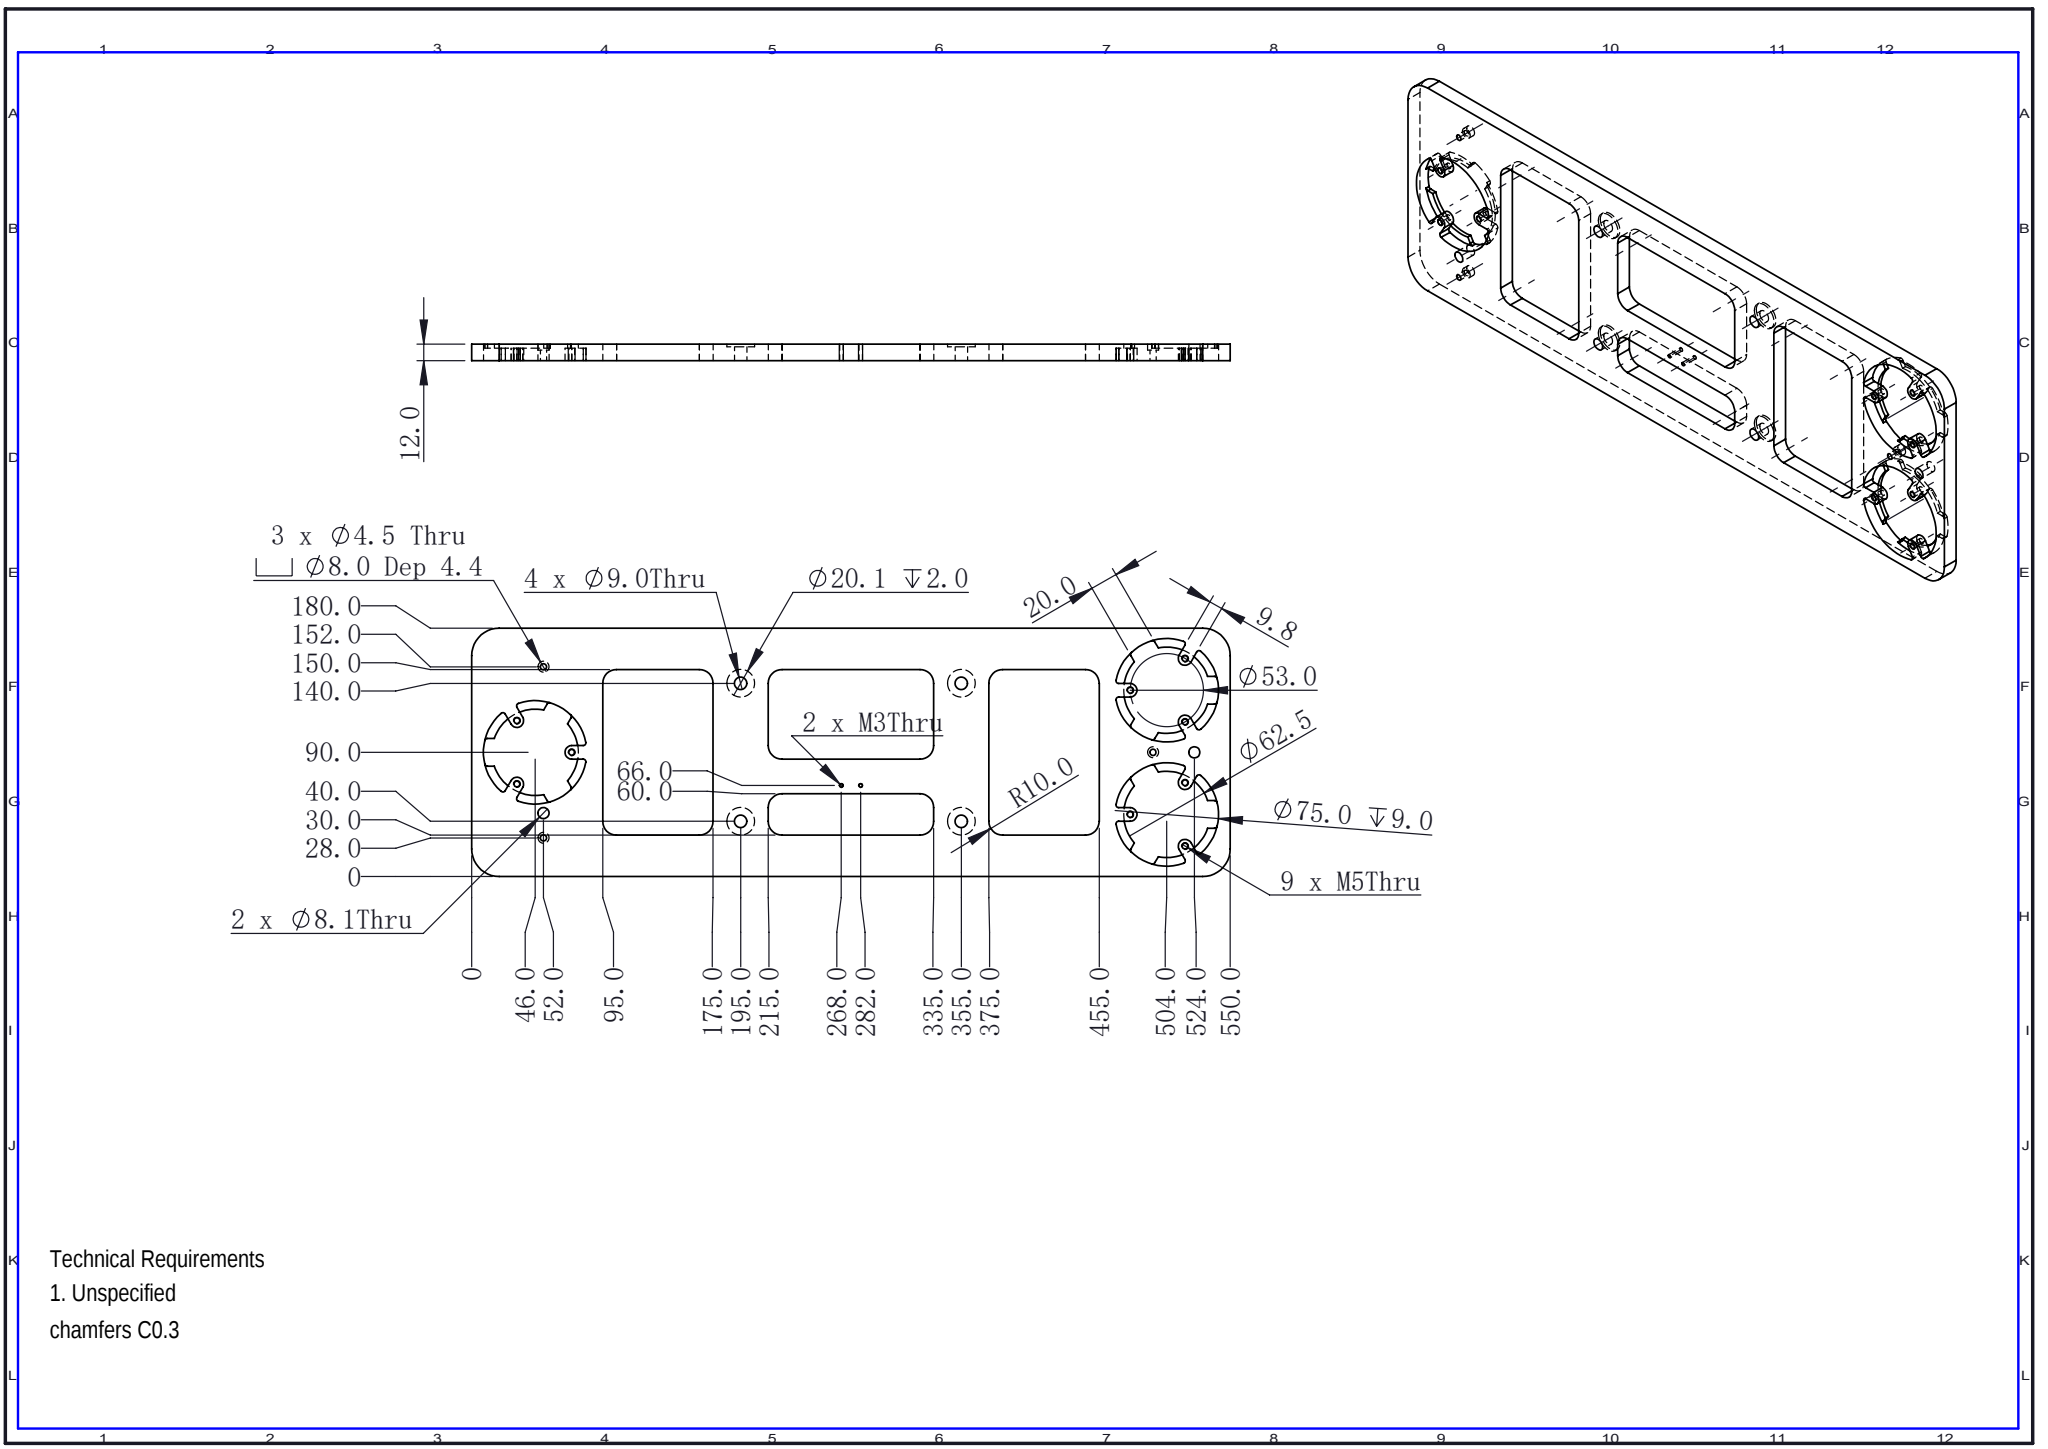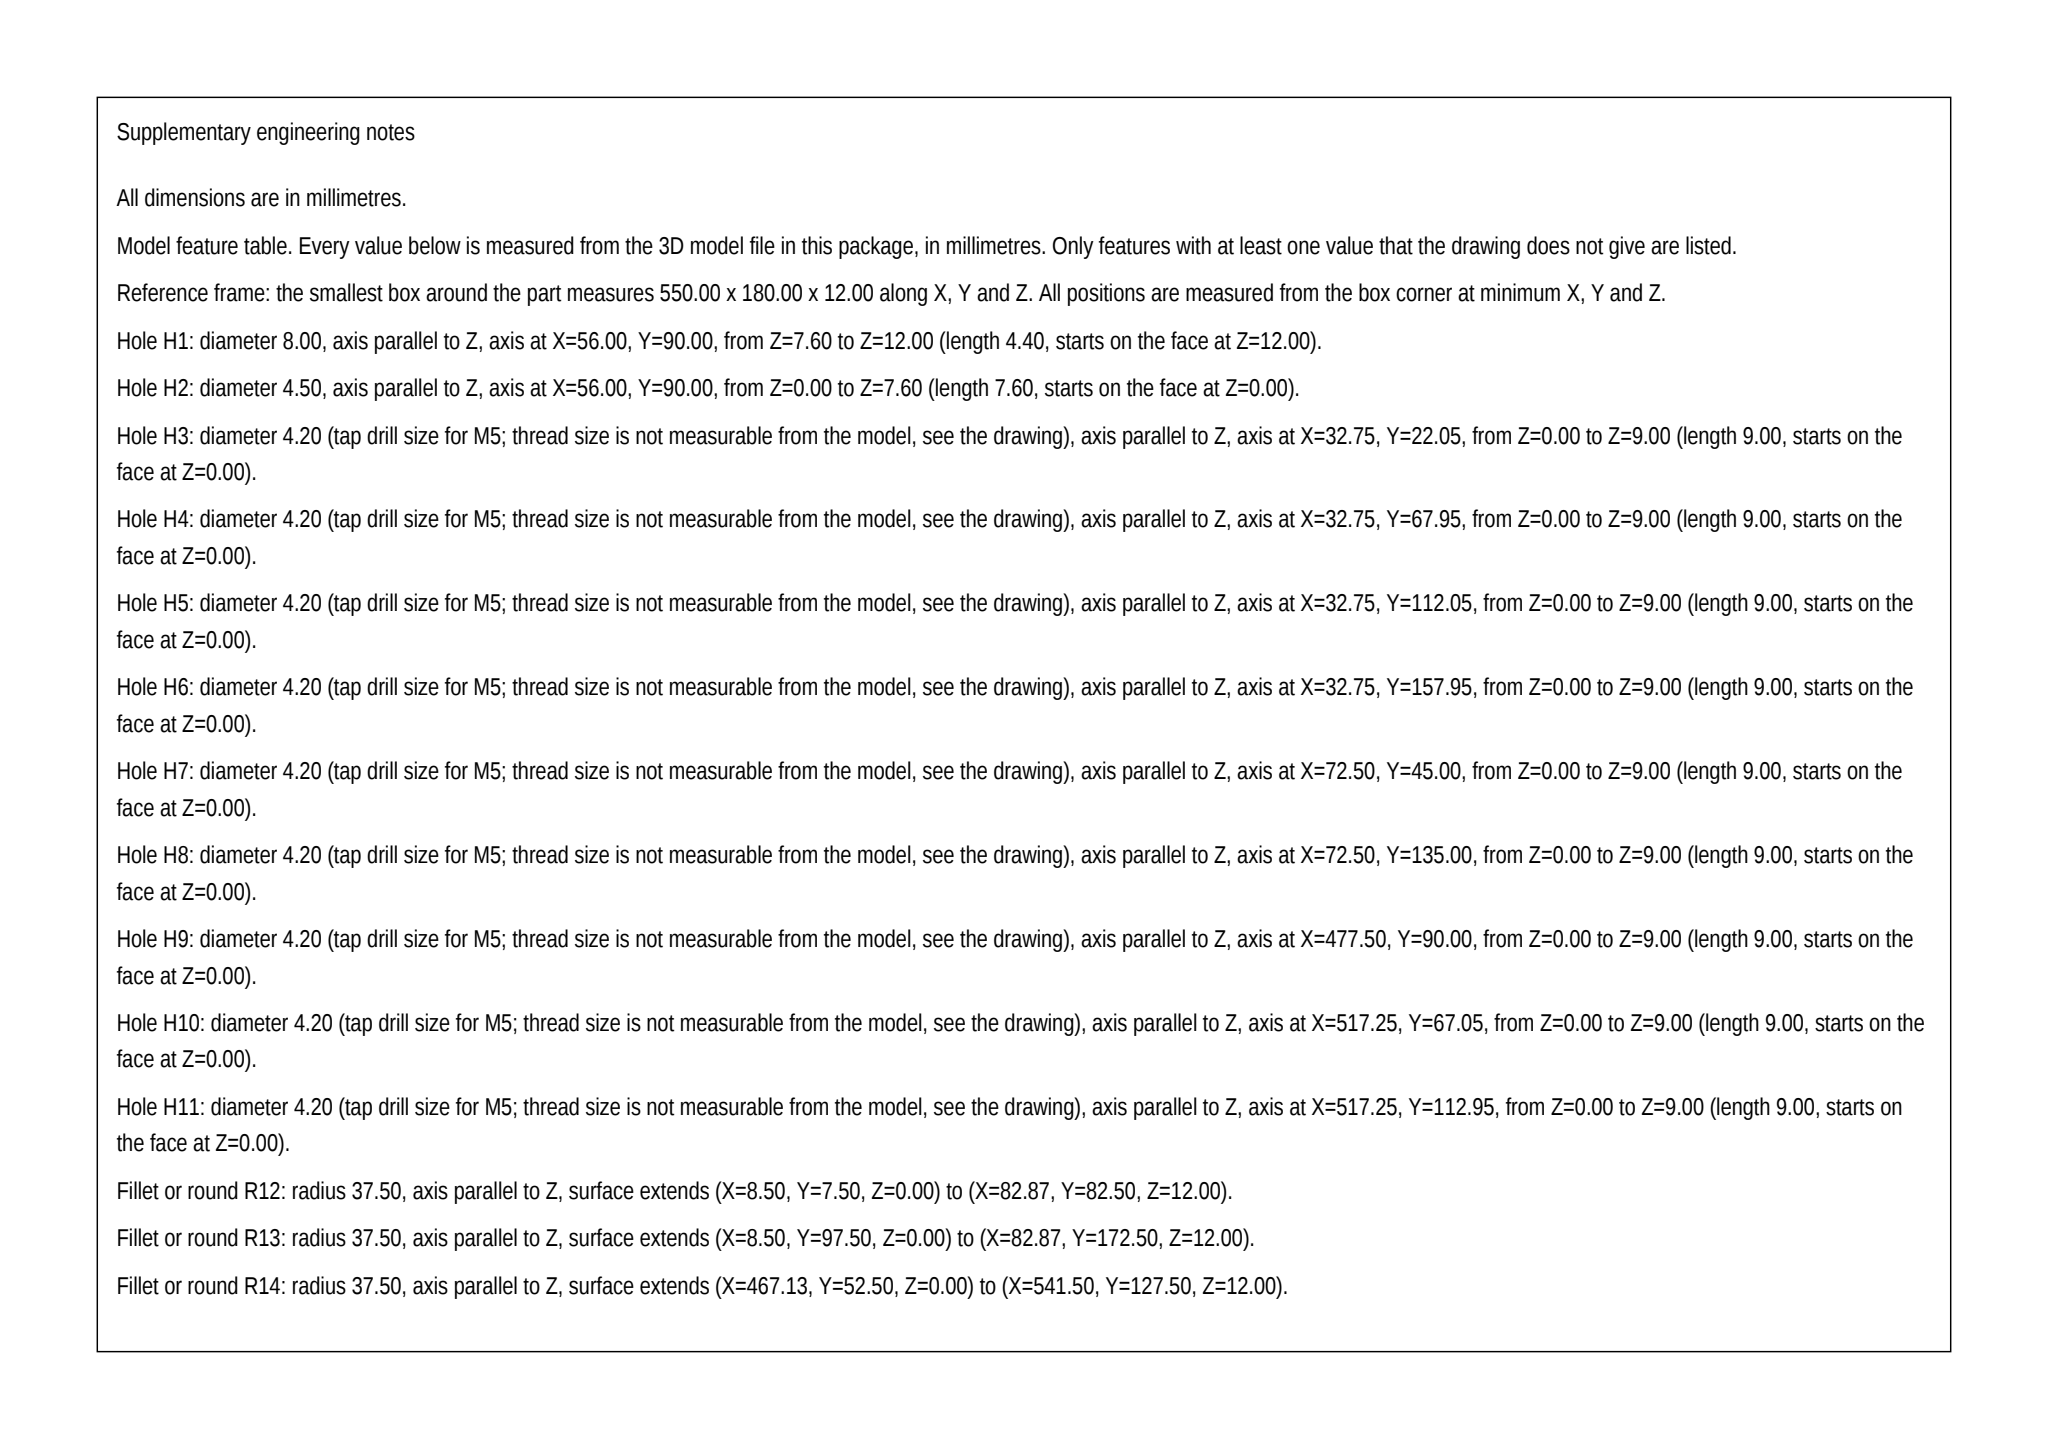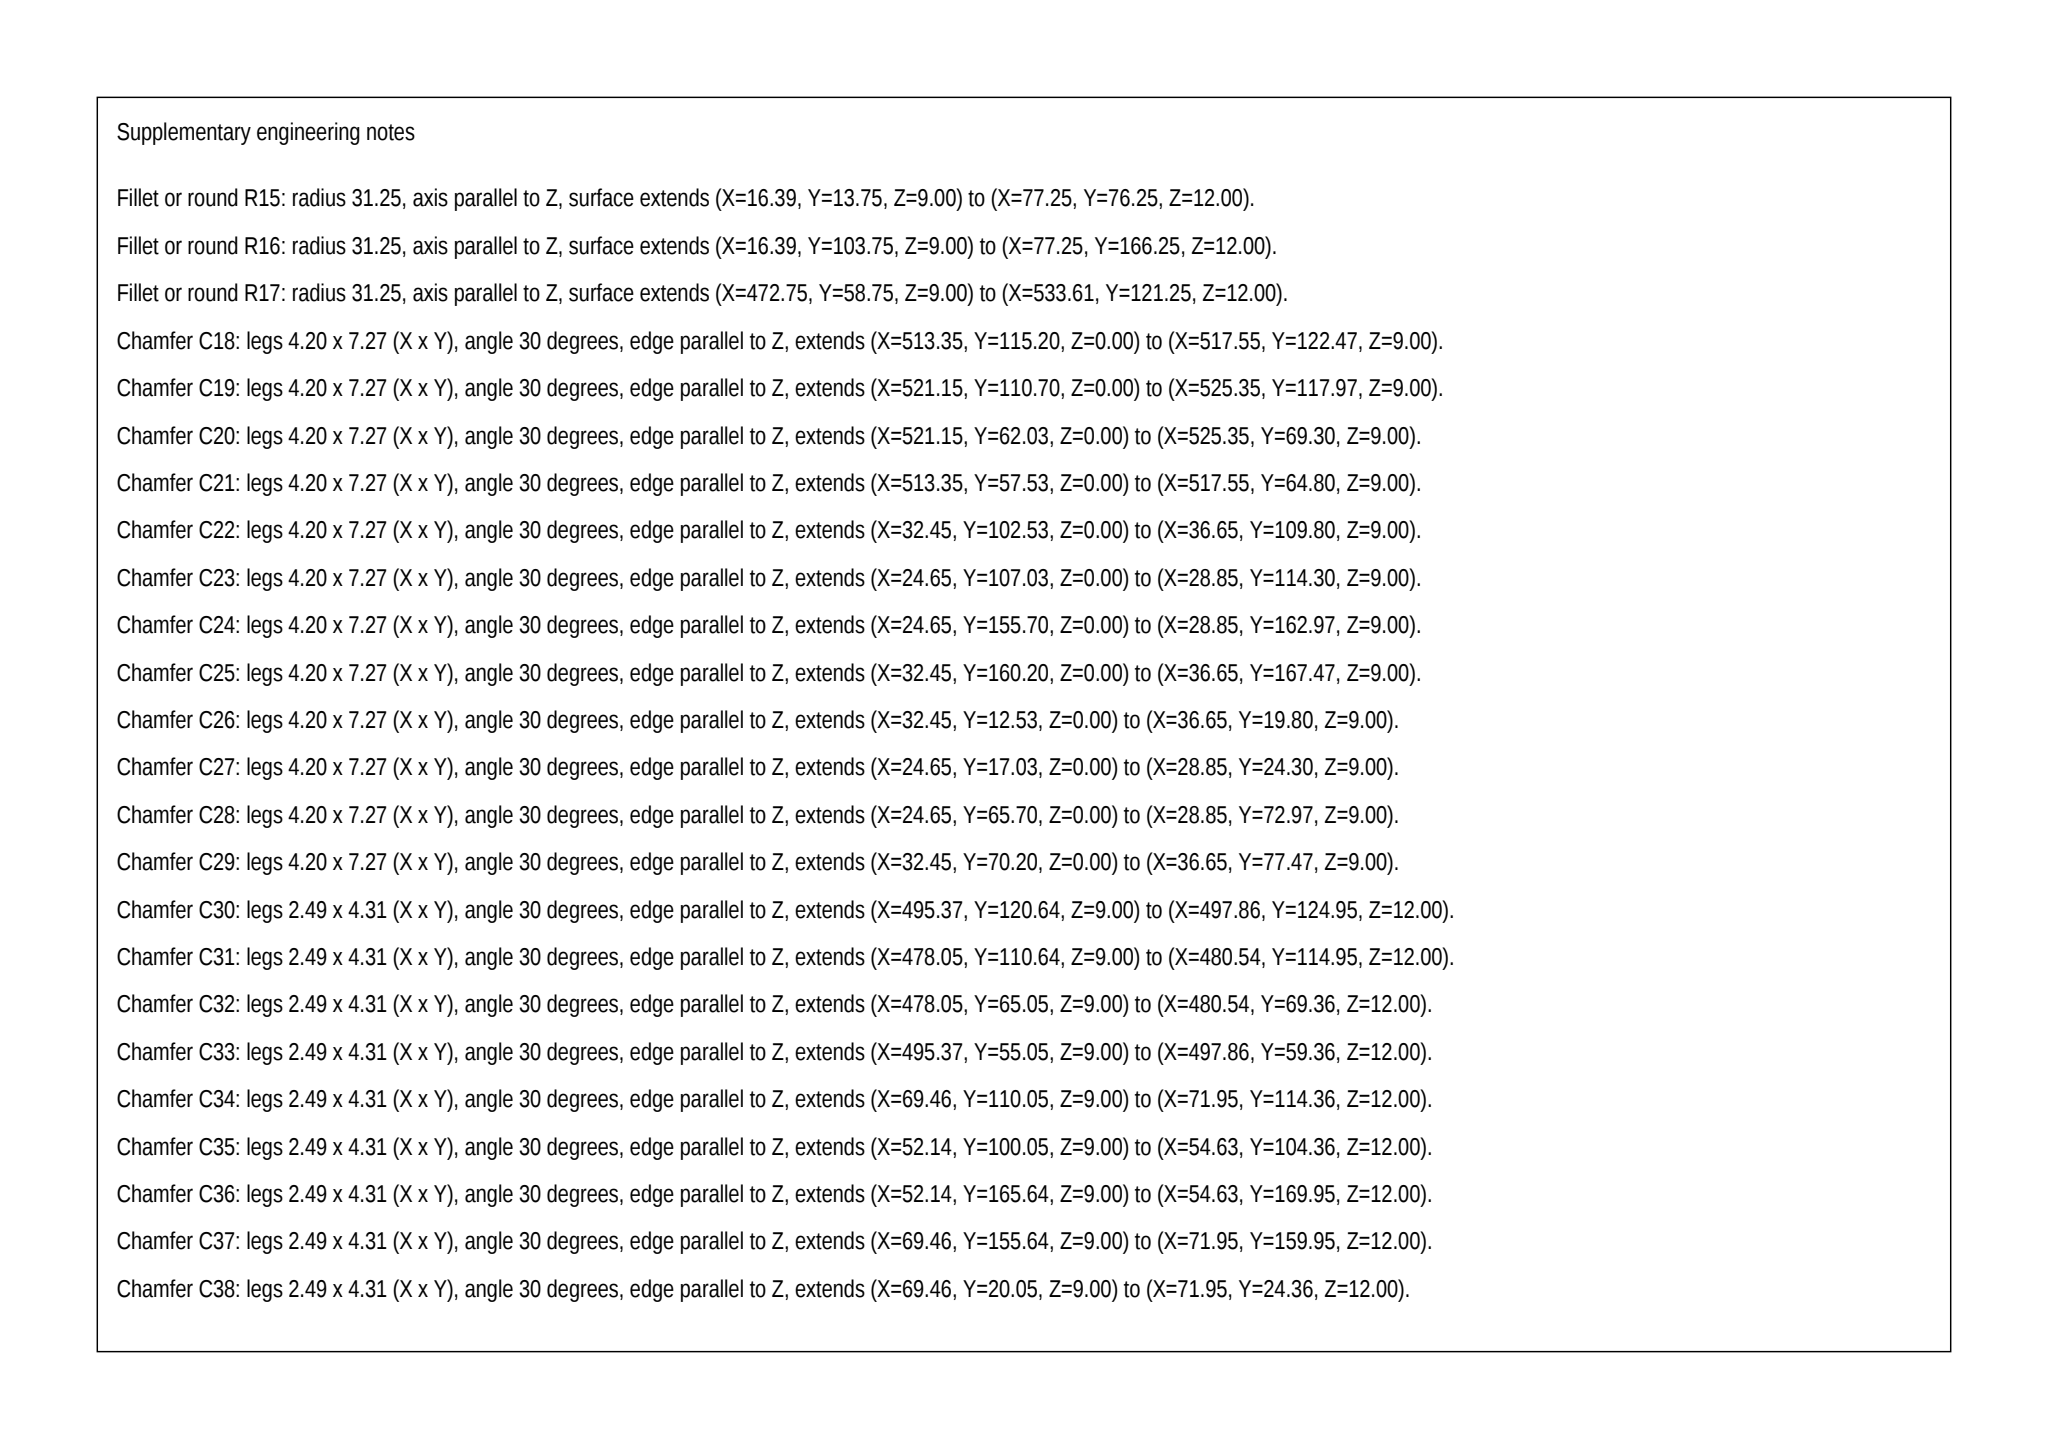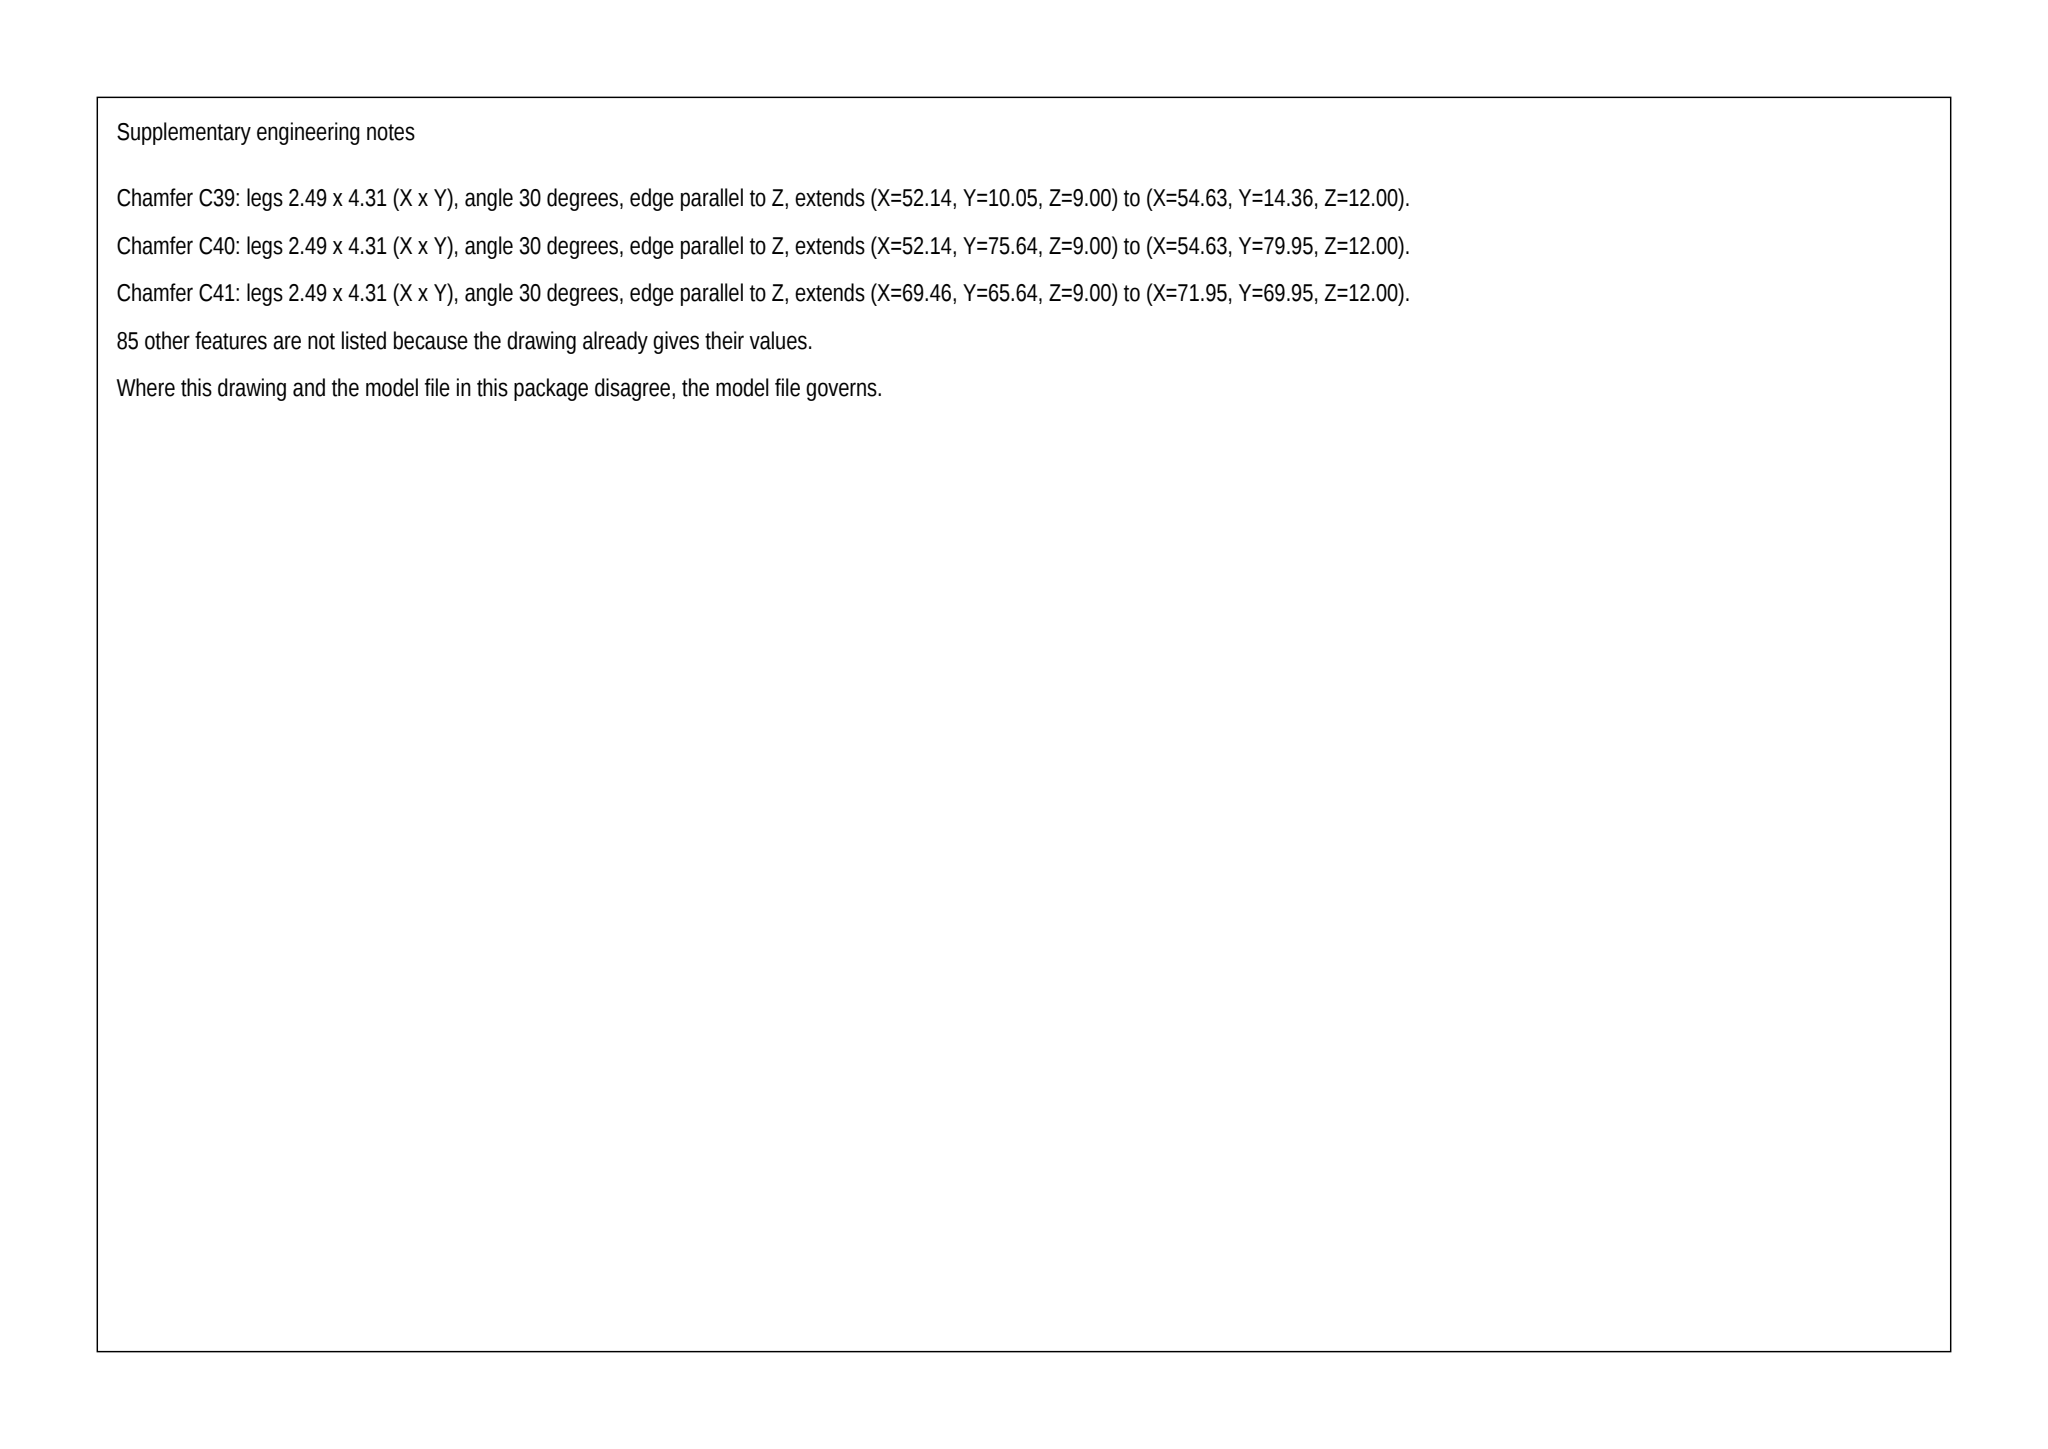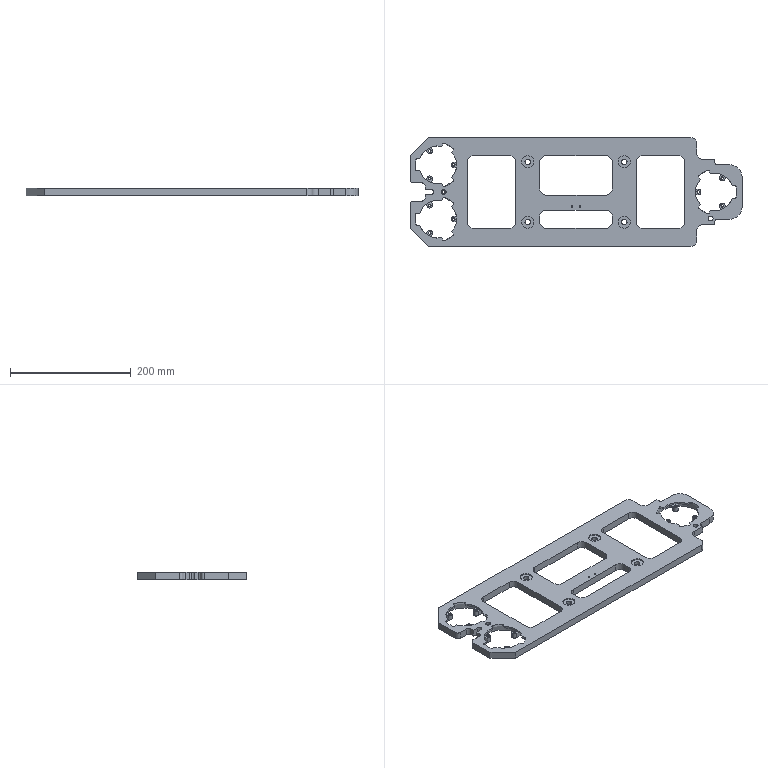Part | SolidWorks | mm | 1 solid | 260 faces | box 550 x 180 x 12 mm | volume 580542 mm3 | cylinder 153 | plane 107 | commonest cylinder face diameters 4 x44 9 x21 20 x20 4.2 x18 75 x11 62.5 x11 20.1 x8 10 x6